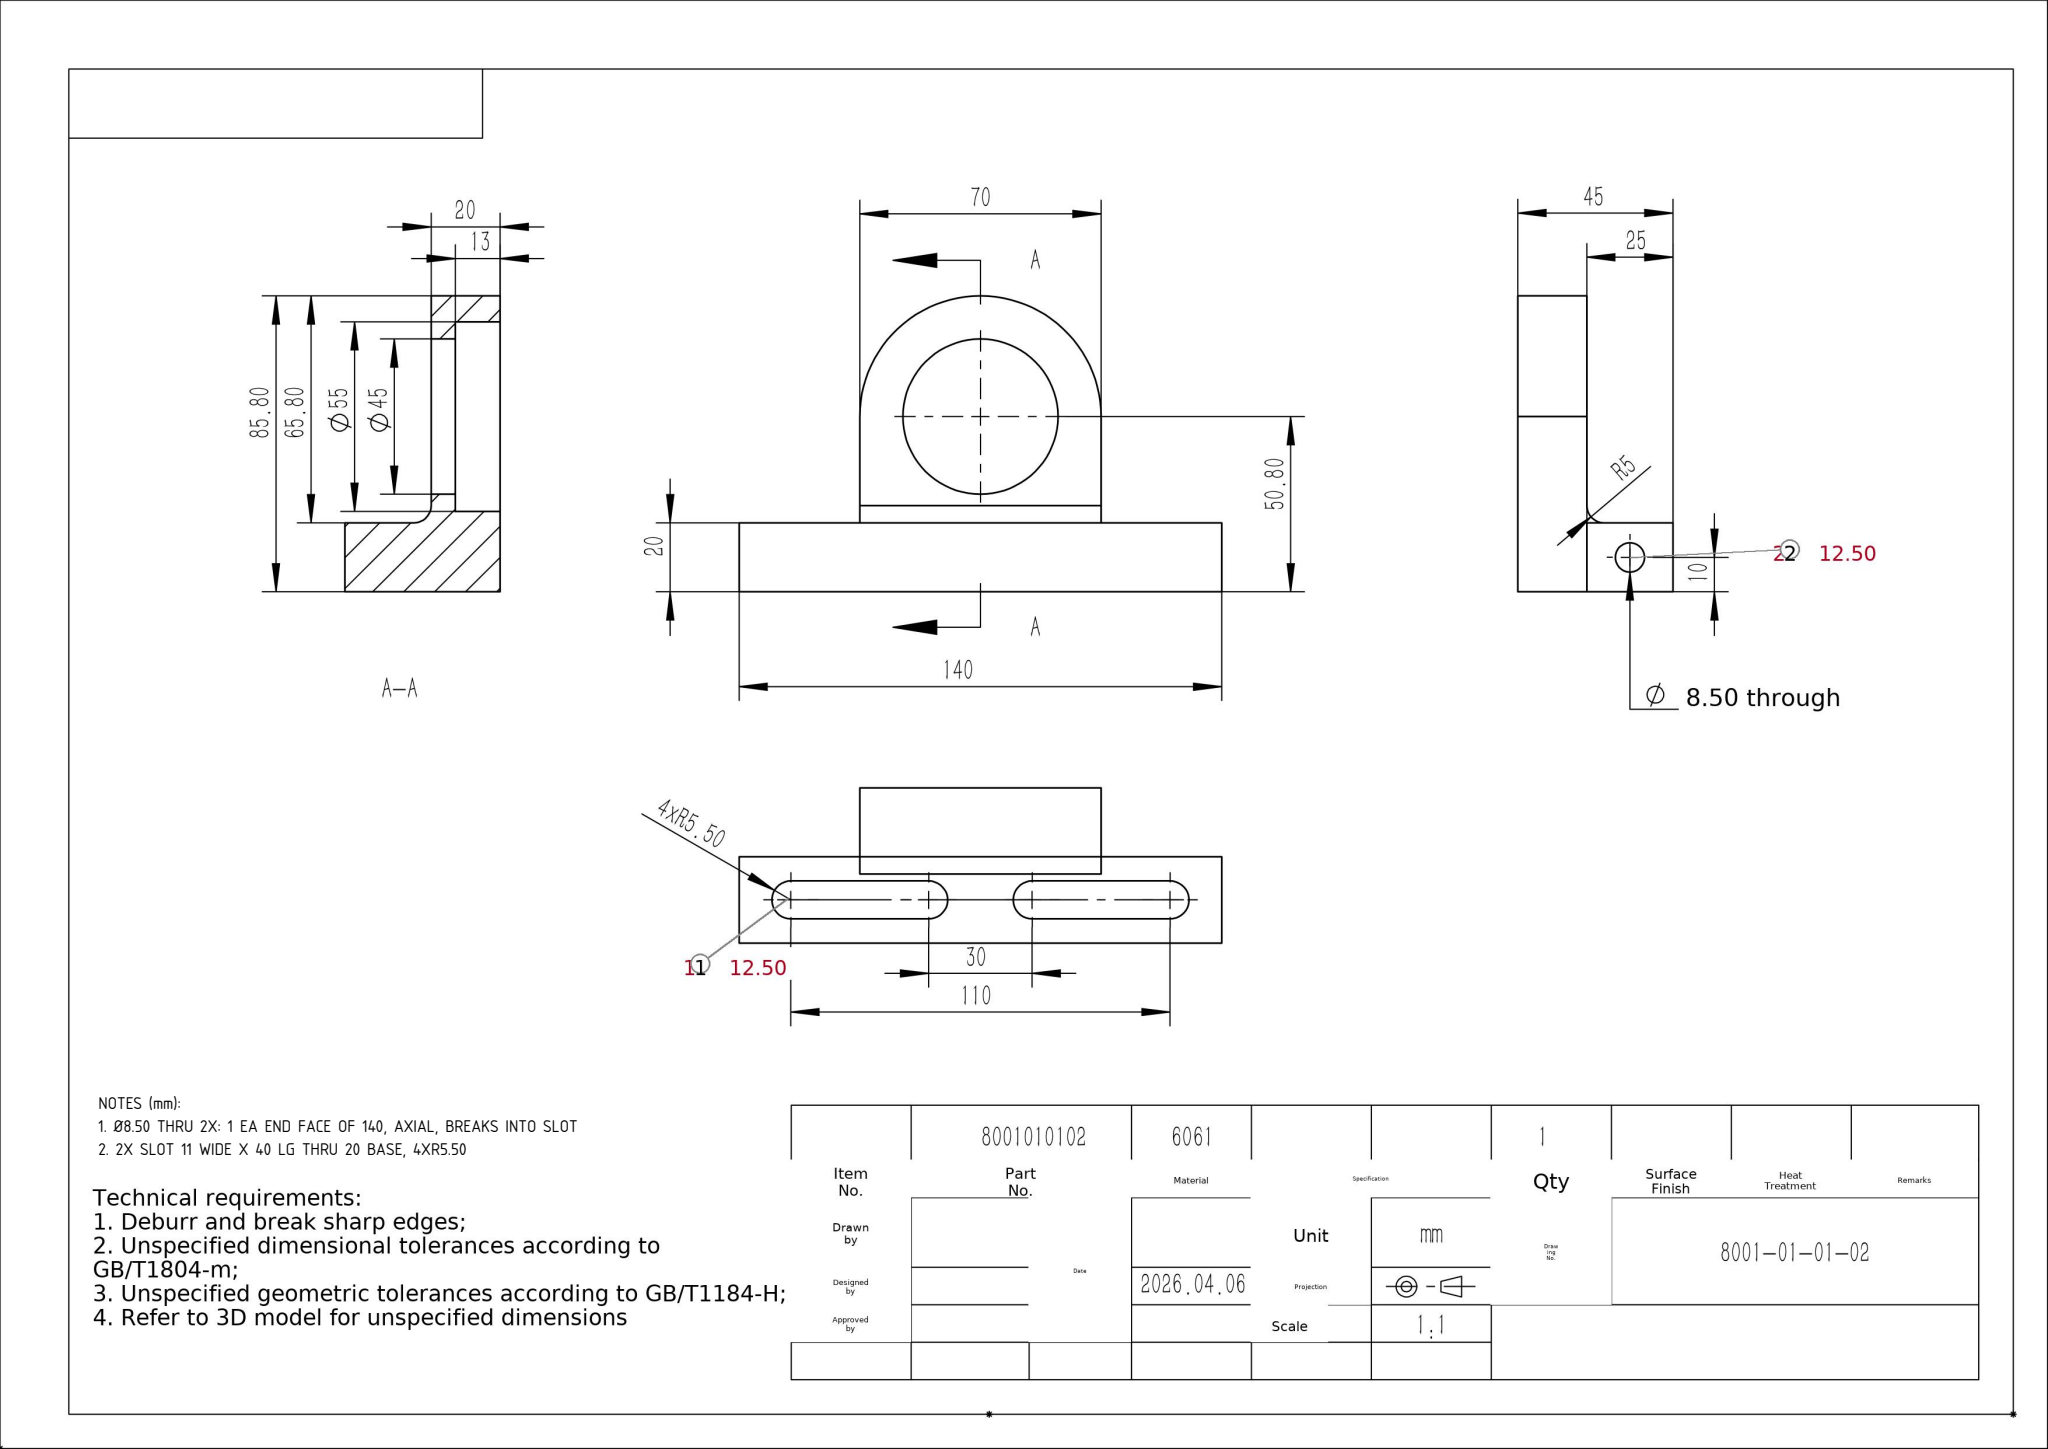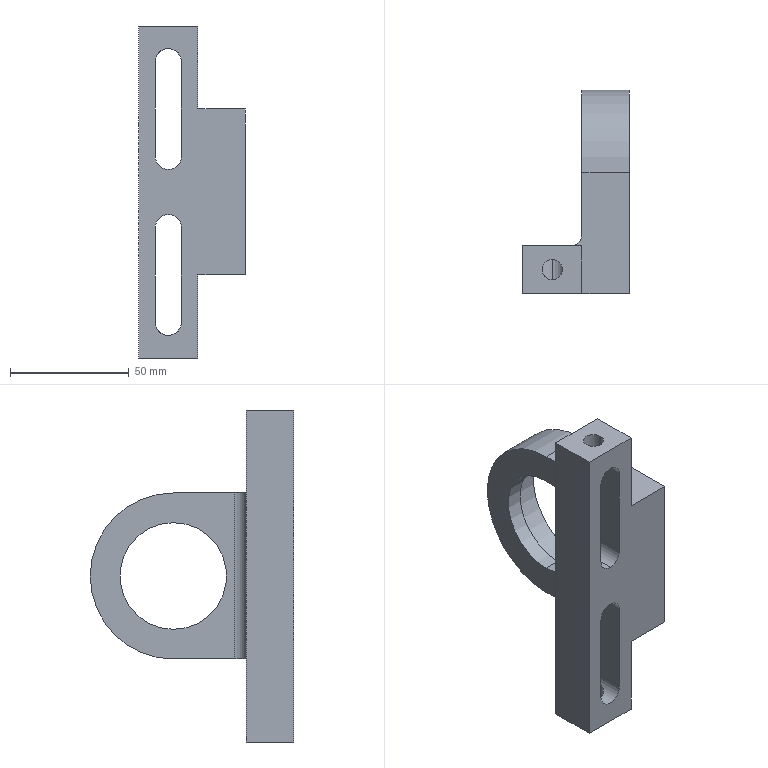Part | SolidWorks | mm | 1 solid | 32 faces | box 45 x 85.8 x 140 mm | volume 115431 mm3 | cylinder 16 | plane 16 | commonest cylinder face diameters 11 x6 8.5 x4 55 x2 45 x2 70 x1 10 x1
Drawing notes:
Ø8.50 THRU 2X: 1 EA END FACE OF 140, AXIAL, BREAKS INTO SLOT | from the solid: cylinders dia 8.5 axis z at [x12.5, y10], len 11.51, count 4 faces = 2 holes, one entering each z=0/z=140 end face; breakout where slot Ø11 (z=15 & z=125) intersects
2X SLOT 11 WIDE X 40 LG THRU 20 BASE, 4XR5.50 | from the solid: 11 dia y-axis cyls, len 20 (= base ht), at x=12.5, z=15&55 and z=85&125 -> two 11-wide slots 40 long thru y=0 to 20
build123d program:
from build123d import *

# Parameters (mm, degrees)
SKETCH1_W                                            = 25
SKETCH1_H                                            = 140
BOSS_EXTRUDE1_DEPTH                                  = 20
BOSS_EXTRUDE2_DEPTH                                  = 20
CUT_EXTRUDE1_DEPTH                                   = 103.248
CUT_EXTRUDE2_DEPTH                                   = 117.132
CYLINDRICAL_COUNTERSUNK_HOLE_FOR_M42_HEX_D           = 45
CYLINDRICAL_COUNTERSUNK_HOLE_FOR_M42_HEX_DEPTH       = 45
CYLINDRICAL_COUNTERSUNK_HOLE_FOR_M42_HEX_CBORE_D     = 55
CYLINDRICAL_COUNTERSUNK_HOLE_FOR_M42_HEX_CBORE_DEPTH = 13
F_8_5_8_5_DIAMETER_HOLE1_REACH                       = 169.889
F_8_5_8_5_DIAMETER_HOLE1_BORE_R                      = 4.25
F_8_5_8_5_DIAMETER_HOLE2_REACH                       = 169.889
F_8_5_8_5_DIAMETER_HOLE2_BORE_R                      = 4.25
FILLET1_R                                            = 5


with BuildPart() as part:
    # Sketch1 → Boss-Extrude1 (new body)
    with BuildSketch(Plane.XZ):
        with Locations((-22.5, 0)):
            Rectangle(SKETCH1_W, SKETCH1_H)
    extrude(amount=-BOSS_EXTRUDE1_DEPTH)

    # Sketch2 → Boss-Extrude2 (add)
    with BuildSketch(Plane(origin=(-10, 0, 0), x_dir=(0, 0, -1), z_dir=(1, 0, 0))):
        with BuildLine():
            Line((35, 0), (-35, 0))
            Line((-35, 0), (-35, 50.8))
            ThreePointArc((-35, 50.8), (0, 85.8), (35, 50.8))
            Line((35, 50.8), (35, 0))
        make_face()
    extrude(amount=BOSS_EXTRUDE2_DEPTH)

    # Sketch3 → Cut-Extrude1 (cut, through all)
    with BuildSketch(Plane(origin=(0, 20, 0), x_dir=(-1, 0, 0), z_dir=(0, 1, 0))):
        with BuildLine():
            Line((17, -15), (17, -55))
            ThreePointArc((17, -55), (22.5, -60.5), (28, -55))
            Line((28, -55), (28, -15))
            ThreePointArc((28, -15), (22.5, -9.5), (17, -15))
        make_face()
    extrude(amount=-CUT_EXTRUDE1_DEPTH, mode=Mode.SUBTRACT)

    # Sketch4 → Cut-Extrude2 (cut, through all)
    with BuildSketch(Plane.XZ):
        with BuildLine():
            Line((-17, 15), (-17, 55))
            ThreePointArc((-17, 55), (-22.5, 60.5), (-28, 55))
            Line((-28, 55), (-28, 15))
            ThreePointArc((-28, 15), (-22.5, 9.5), (-17, 15))
        make_face()
    extrude(amount=-CUT_EXTRUDE2_DEPTH, mode=Mode.SUBTRACT)

    # Cylindrical Countersunk Hole for M42 Hex
    with Locations(Plane(origin=(10, 0, 0), x_dir=(0, 0, -1), z_dir=(1, 0, 0))):
        with Locations((0, 50.8)):
            CounterBoreHole(CYLINDRICAL_COUNTERSUNK_HOLE_FOR_M42_HEX_D / 2, CYLINDRICAL_COUNTERSUNK_HOLE_FOR_M42_HEX_CBORE_D / 2, CYLINDRICAL_COUNTERSUNK_HOLE_FOR_M42_HEX_CBORE_DEPTH, depth=CYLINDRICAL_COUNTERSUNK_HOLE_FOR_M42_HEX_DEPTH)

    # 8.5 _8.5_ Diameter Hole1 bore → 8.5 _8.5_ Diameter Hole1 (cut, up to next)
    with BuildSketch(Plane(origin=(0, 0, -70), x_dir=(-1, 0, 0), z_dir=(0, 0, -1)), mode=Mode.PRIVATE) as f_8_5_8_5_diameter_hole1_sk1:
        with Locations((22.5, 10)):
            Circle(F_8_5_8_5_DIAMETER_HOLE1_BORE_R)
    f_8_5_8_5_diameter_hole1_tool1 = extrude(f_8_5_8_5_diameter_hole1_sk1.sketch, amount=-F_8_5_8_5_DIAMETER_HOLE1_REACH, mode=Mode.PRIVATE) & part.part
    add(f_8_5_8_5_diameter_hole1_tool1.solids().sort_by_distance((-22.5, 10, -70))[0], mode=Mode.SUBTRACT)

    # 8.5 _8.5_ Diameter Hole2 bore → 8.5 _8.5_ Diameter Hole2 (cut, up to next)
    with BuildSketch(Plane.XY.offset(70), mode=Mode.PRIVATE) as f_8_5_8_5_diameter_hole2_sk1:
        with Locations((-22.5, 10)):
            Circle(F_8_5_8_5_DIAMETER_HOLE2_BORE_R)
    f_8_5_8_5_diameter_hole2_tool1 = extrude(f_8_5_8_5_diameter_hole2_sk1.sketch, amount=-F_8_5_8_5_DIAMETER_HOLE2_REACH, mode=Mode.PRIVATE) & part.part
    add(f_8_5_8_5_diameter_hole2_tool1.solids().sort_by_distance((-22.5, 10, 70))[0], mode=Mode.SUBTRACT)

    # Fillet1
    fillet1_edges = [part.edges().sort_by_distance(p)[0] for p in [
        (-10, 20, 0),
    ]]
    fillet(fillet1_edges, radius=FILLET1_R)


solid = part.part